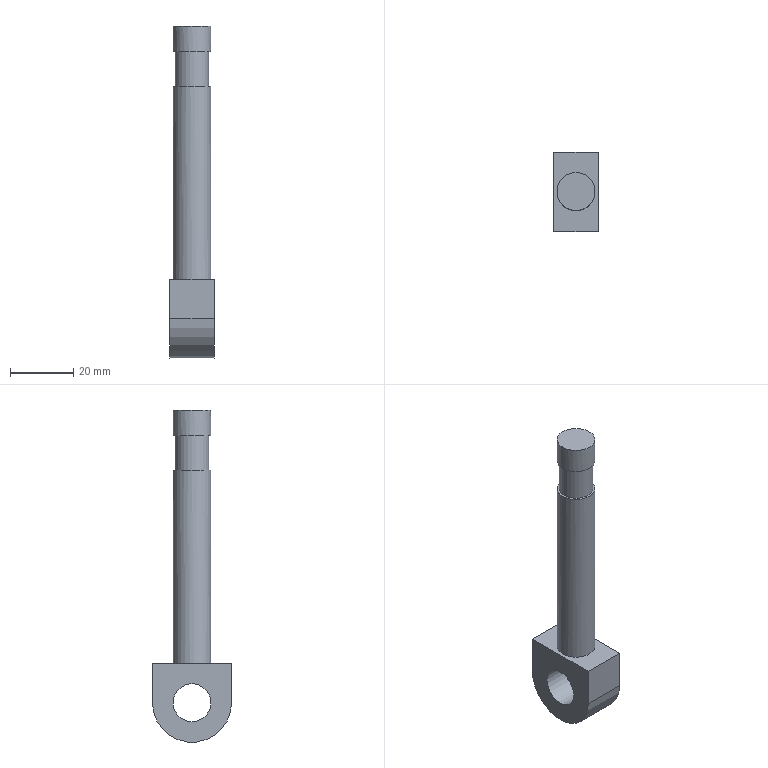Component | NX | HINGE_SCREW | 1 solid | 13 faces | box 14 x 25 x 105 mm | volume 15003 mm3 | plane 8 | cylinder 5 | commonest cylinder face diameters 12 x3 25 x1 10.579 x1
STEP:
#1=CARTESIAN_POINT('',(0.,0.,0.));
#2=DIRECTION('',(0.,0.,1.));
#3=DIRECTION('',(1.,0.,0.));
#4=AXIS2_PLACEMENT_3D('',#1,#2,#3);
#5=CARTESIAN_POINT('',(553.625,-108.409,-19.557));
#6=VERTEX_POINT('',#5);
#7=CARTESIAN_POINT('',(553.625,-108.409,-32.057));
#8=VERTEX_POINT('',#7);
#9=CARTESIAN_POINT('',(553.625,-108.409,-19.557));
#10=DIRECTION('',(0.,0.,-1.));
#11=VECTOR('',#10,1.);
#12=LINE('',#9,#11);
#13=CARTESIAN_POINT('',(567.625,-108.409,-19.557));
#14=DIRECTION('',(0.,1.,0.));
#15=DIRECTION('',(0.,0.,1.));
#16=AXIS2_PLACEMENT_3D('',#13,#14,#15);
#17=PLANE('',#16);
#18=CARTESIAN_POINT('',(0.,-14.));
#19=DIRECTION('',(-1.,0.));
#20=VECTOR('',#19,1.);
#21=LINE('',#18,#20);
#22=(GEOMETRIC_REPRESENTATION_CONTEXT(2)PARAMETRIC_REPRESENTATION_CONTEXT()REPRESENTATION_CONTEXT('',''));
#23=DEFINITIONAL_REPRESENTATION('',(#21),#22);
#24=PCURVE('',#17,#23);
#25=CARTESIAN_POINT('',(553.625,-95.909,-32.057));
#26=DIRECTION('',(1.,0.,0.));
#27=DIRECTION('',(0.,0.,-1.));
#28=AXIS2_PLACEMENT_3D('',#25,#26,#27);
#29=PLANE('',#28);
#30=CARTESIAN_POINT('',(-12.5,-12.5));
#31=DIRECTION('',(1.,0.));
#32=VECTOR('',#31,1.);
#33=LINE('',#30,#32);
#34=(GEOMETRIC_REPRESENTATION_CONTEXT(2)PARAMETRIC_REPRESENTATION_CONTEXT()REPRESENTATION_CONTEXT('',''));
#35=DEFINITIONAL_REPRESENTATION('',(#33),#34);
#36=PCURVE('',#29,#35);
#37=SURFACE_CURVE('',#12,(#24,#36),.PCURVE_S1.);
#38=EDGE_CURVE('',#6,#8,#37,.T.);
#39=ORIENTED_EDGE('',*,*,#38,.T.);
#40=CARTESIAN_POINT('',(567.625,-108.409,-32.057));
#41=VERTEX_POINT('',#40);
#42=CARTESIAN_POINT('',(567.625,-108.409,-32.057));
#43=DIRECTION('',(-1.,0.,0.));
#44=VECTOR('',#43,1.);
#45=LINE('',#42,#44);
#46=CARTESIAN_POINT('',(-12.5,0.));
#47=DIRECTION('',(0.,-1.));
#48=VECTOR('',#47,1.);
#49=LINE('',#46,#48);
#50=(GEOMETRIC_REPRESENTATION_CONTEXT(2)PARAMETRIC_REPRESENTATION_CONTEXT()REPRESENTATION_CONTEXT('',''));
#51=DEFINITIONAL_REPRESENTATION('',(#49),#50);
#52=PCURVE('',#17,#51);
#53=CARTESIAN_POINT('',(567.625,-95.909,-32.057));
#54=DIRECTION('',(-1.,0.,0.));
#55=DIRECTION('',(0.,0.,1.));
#56=AXIS2_PLACEMENT_3D('',#53,#54,#55);
#57=CYLINDRICAL_SURFACE('',#56,12.5);
#58=CARTESIAN_POINT('',(4.712,0.));
#59=DIRECTION('',(0.,1.));
#60=VECTOR('',#59,1.);
#61=LINE('',#58,#60);
#62=(GEOMETRIC_REPRESENTATION_CONTEXT(2)PARAMETRIC_REPRESENTATION_CONTEXT()REPRESENTATION_CONTEXT('',''));
#63=DEFINITIONAL_REPRESENTATION('',(#61),#62);
#64=PCURVE('',#57,#63);
#65=SURFACE_CURVE('',#45,(#52,#64),.PCURVE_S1.);
#66=EDGE_CURVE('',#41,#8,#65,.T.);
#67=ORIENTED_EDGE('',*,*,#66,.F.);
#68=CARTESIAN_POINT('',(567.625,-108.409,-19.557));
#69=VERTEX_POINT('',#68);
#70=CARTESIAN_POINT('',(567.625,-108.409,-19.557));
#71=DIRECTION('',(0.,0.,-1.));
#72=VECTOR('',#71,1.);
#73=LINE('',#70,#72);
#74=CARTESIAN_POINT('',(0.,0.));
#75=DIRECTION('',(-1.,0.));
#76=VECTOR('',#75,1.);
#77=LINE('',#74,#76);
#78=(GEOMETRIC_REPRESENTATION_CONTEXT(2)PARAMETRIC_REPRESENTATION_CONTEXT()REPRESENTATION_CONTEXT('',''));
#79=DEFINITIONAL_REPRESENTATION('',(#77),#78);
#80=PCURVE('',#17,#79);
#81=CARTESIAN_POINT('',(567.625,-95.909,-32.057));
#82=DIRECTION('',(1.,0.,0.));
#83=DIRECTION('',(0.,0.,-1.));
#84=AXIS2_PLACEMENT_3D('',#81,#82,#83);
#85=PLANE('',#84);
#86=CARTESIAN_POINT('',(-12.5,-12.5));
#87=DIRECTION('',(1.,0.));
#88=VECTOR('',#87,1.);
#89=LINE('',#86,#88);
#90=(GEOMETRIC_REPRESENTATION_CONTEXT(2)PARAMETRIC_REPRESENTATION_CONTEXT()REPRESENTATION_CONTEXT('',''));
#91=DEFINITIONAL_REPRESENTATION('',(#89),#90);
#92=PCURVE('',#85,#91);
#93=SURFACE_CURVE('',#73,(#80,#92),.PCURVE_S1.);
#94=EDGE_CURVE('',#69,#41,#93,.T.);
#95=ORIENTED_EDGE('',*,*,#94,.F.);
#96=CARTESIAN_POINT('',(567.625,-108.409,-19.557));
#97=DIRECTION('',(-1.,0.,0.));
#98=VECTOR('',#97,1.);
#99=LINE('',#96,#98);
#100=CARTESIAN_POINT('',(0.,0.));
#101=DIRECTION('',(0.,-1.));
#102=VECTOR('',#101,1.);
#103=LINE('',#100,#102);
#104=(GEOMETRIC_REPRESENTATION_CONTEXT(2)PARAMETRIC_REPRESENTATION_CONTEXT()REPRESENTATION_CONTEXT('',''));
#105=DEFINITIONAL_REPRESENTATION('',(#103),#104);
#106=PCURVE('',#17,#105);
#107=CARTESIAN_POINT('',(567.625,-83.409,-19.557));
#108=DIRECTION('',(0.,0.,-1.));
#109=DIRECTION('',(0.,1.,0.));
#110=AXIS2_PLACEMENT_3D('',#107,#108,#109);
#111=PLANE('',#110);
#112=CARTESIAN_POINT('',(-25.,0.));
#113=DIRECTION('',(0.,-1.));
#114=VECTOR('',#113,1.);
#115=LINE('',#112,#114);
#116=(GEOMETRIC_REPRESENTATION_CONTEXT(2)PARAMETRIC_REPRESENTATION_CONTEXT()REPRESENTATION_CONTEXT('',''));
#117=DEFINITIONAL_REPRESENTATION('',(#115),#116);
#118=PCURVE('',#111,#117);
#119=SURFACE_CURVE('',#99,(#106,#118),.PCURVE_S1.);
#120=EDGE_CURVE('',#69,#6,#119,.T.);
#121=ORIENTED_EDGE('',*,*,#120,.T.);
#122=EDGE_LOOP('',(#39,#67,#95,#121));
#123=FACE_BOUND('',#122,.T.);
#124=ADVANCED_FACE('',(#123),#17,.F.);
#125=CARTESIAN_POINT('',(553.625,-83.409,-32.057));
#126=VERTEX_POINT('',#125);
#127=CARTESIAN_POINT('',(553.625,-95.909,-32.057));
#128=DIRECTION('',(1.,0.,0.));
#129=DIRECTION('',(0.,1.,0.));
#130=AXIS2_PLACEMENT_3D('',#127,#128,#129);
#131=CIRCLE('',#130,12.5);
#132=CARTESIAN_POINT('',(7.854,14.));
#133=DIRECTION('',(-1.,0.));
#134=VECTOR('',#133,1.);
#135=LINE('',#132,#134);
#136=(GEOMETRIC_REPRESENTATION_CONTEXT(2)PARAMETRIC_REPRESENTATION_CONTEXT()REPRESENTATION_CONTEXT('',''));
#137=DEFINITIONAL_REPRESENTATION('',(#135),#136);
#138=PCURVE('',#57,#137);
#139=CARTESIAN_POINT('',(0.,0.));
#140=DIRECTION('',(0.,1.));
#141=AXIS2_PLACEMENT_2D('',#139,#140);
#142=CIRCLE('',#141,12.5);
#143=(GEOMETRIC_REPRESENTATION_CONTEXT(2)PARAMETRIC_REPRESENTATION_CONTEXT()REPRESENTATION_CONTEXT('',''));
#144=DEFINITIONAL_REPRESENTATION('',(#142),#143);
#145=PCURVE('',#29,#144);
#146=SURFACE_CURVE('',#131,(#138,#145),.PCURVE_S1.);
#147=EDGE_CURVE('',#8,#126,#146,.T.);
#148=ORIENTED_EDGE('',*,*,#147,.T.);
#149=CARTESIAN_POINT('',(567.625,-83.409,-32.057));
#150=VERTEX_POINT('',#149);
#151=CARTESIAN_POINT('',(567.625,-83.409,-32.057));
#152=DIRECTION('',(-1.,0.,0.));
#153=VECTOR('',#152,1.);
#154=LINE('',#151,#153);
#155=CARTESIAN_POINT('',(1.571,0.));
#156=DIRECTION('',(0.,1.));
#157=VECTOR('',#156,1.);
#158=LINE('',#155,#157);
#159=(GEOMETRIC_REPRESENTATION_CONTEXT(2)PARAMETRIC_REPRESENTATION_CONTEXT()REPRESENTATION_CONTEXT('',''));
#160=DEFINITIONAL_REPRESENTATION('',(#158),#159);
#161=PCURVE('',#57,#160);
#162=CARTESIAN_POINT('',(567.625,-83.409,-32.057));
#163=DIRECTION('',(0.,-1.,0.));
#164=DIRECTION('',(0.,0.,-1.));
#165=AXIS2_PLACEMENT_3D('',#162,#163,#164);
#166=PLANE('',#165);
#167=CARTESIAN_POINT('',(0.,0.));
#168=DIRECTION('',(0.,-1.));
#169=VECTOR('',#168,1.);
#170=LINE('',#167,#169);
#171=(GEOMETRIC_REPRESENTATION_CONTEXT(2)PARAMETRIC_REPRESENTATION_CONTEXT()REPRESENTATION_CONTEXT('',''));
#172=DEFINITIONAL_REPRESENTATION('',(#170),#171);
#173=PCURVE('',#166,#172);
#174=SURFACE_CURVE('',#154,(#161,#173),.PCURVE_S1.);
#175=EDGE_CURVE('',#150,#126,#174,.T.);
#176=ORIENTED_EDGE('',*,*,#175,.F.);
#177=CARTESIAN_POINT('',(567.625,-95.909,-32.057));
#178=DIRECTION('',(1.,0.,0.));
#179=DIRECTION('',(0.,1.,0.));
#180=AXIS2_PLACEMENT_3D('',#177,#178,#179);
#181=CIRCLE('',#180,12.5);
#182=CARTESIAN_POINT('',(7.854,0.));
#183=DIRECTION('',(-1.,0.));
#184=VECTOR('',#183,1.);
#185=LINE('',#182,#184);
#186=(GEOMETRIC_REPRESENTATION_CONTEXT(2)PARAMETRIC_REPRESENTATION_CONTEXT()REPRESENTATION_CONTEXT('',''));
#187=DEFINITIONAL_REPRESENTATION('',(#185),#186);
#188=PCURVE('',#57,#187);
#189=CARTESIAN_POINT('',(0.,0.));
#190=DIRECTION('',(0.,1.));
#191=AXIS2_PLACEMENT_2D('',#189,#190);
#192=CIRCLE('',#191,12.5);
#193=(GEOMETRIC_REPRESENTATION_CONTEXT(2)PARAMETRIC_REPRESENTATION_CONTEXT()REPRESENTATION_CONTEXT('',''));
#194=DEFINITIONAL_REPRESENTATION('',(#192),#193);
#195=PCURVE('',#85,#194);
#196=SURFACE_CURVE('',#181,(#188,#195),.PCURVE_S1.);
#197=EDGE_CURVE('',#41,#150,#196,.T.);
#198=ORIENTED_EDGE('',*,*,#197,.F.);
#199=ORIENTED_EDGE('',*,*,#66,.T.);
#200=EDGE_LOOP('',(#148,#176,#198,#199));
#201=FACE_BOUND('',#200,.T.);
#202=ADVANCED_FACE('',(#201),#57,.T.);
#203=CARTESIAN_POINT('',(553.625,-83.409,-19.557));
#204=VERTEX_POINT('',#203);
#205=CARTESIAN_POINT('',(553.625,-83.409,-32.057));
#206=DIRECTION('',(0.,0.,1.));
#207=VECTOR('',#206,1.);
#208=LINE('',#205,#207);
#209=CARTESIAN_POINT('',(0.,-14.));
#210=DIRECTION('',(-1.,0.));
#211=VECTOR('',#210,1.);
#212=LINE('',#209,#211);
#213=(GEOMETRIC_REPRESENTATION_CONTEXT(2)PARAMETRIC_REPRESENTATION_CONTEXT()REPRESENTATION_CONTEXT('',''));
#214=DEFINITIONAL_REPRESENTATION('',(#212),#213);
#215=PCURVE('',#166,#214);
#216=CARTESIAN_POINT('',(0.,12.5));
#217=DIRECTION('',(-1.,0.));
#218=VECTOR('',#217,1.);
#219=LINE('',#216,#218);
#220=(GEOMETRIC_REPRESENTATION_CONTEXT(2)PARAMETRIC_REPRESENTATION_CONTEXT()REPRESENTATION_CONTEXT('',''));
#221=DEFINITIONAL_REPRESENTATION('',(#219),#220);
#222=PCURVE('',#29,#221);
#223=SURFACE_CURVE('',#208,(#215,#222),.PCURVE_S1.);
#224=EDGE_CURVE('',#126,#204,#223,.T.);
#225=ORIENTED_EDGE('',*,*,#224,.T.);
#226=CARTESIAN_POINT('',(567.625,-83.409,-19.557));
#227=VERTEX_POINT('',#226);
#228=CARTESIAN_POINT('',(567.625,-83.409,-19.557));
#229=DIRECTION('',(-1.,0.,0.));
#230=VECTOR('',#229,1.);
#231=LINE('',#228,#230);
#232=CARTESIAN_POINT('',(-12.5,0.));
#233=DIRECTION('',(0.,-1.));
#234=VECTOR('',#233,1.);
#235=LINE('',#232,#234);
#236=(GEOMETRIC_REPRESENTATION_CONTEXT(2)PARAMETRIC_REPRESENTATION_CONTEXT()REPRESENTATION_CONTEXT('',''));
#237=DEFINITIONAL_REPRESENTATION('',(#235),#236);
#238=PCURVE('',#166,#237);
#239=CARTESIAN_POINT('',(0.,0.));
#240=DIRECTION('',(0.,-1.));
#241=VECTOR('',#240,1.);
#242=LINE('',#239,#241);
#243=(GEOMETRIC_REPRESENTATION_CONTEXT(2)PARAMETRIC_REPRESENTATION_CONTEXT()REPRESENTATION_CONTEXT('',''));
#244=DEFINITIONAL_REPRESENTATION('',(#242),#243);
#245=PCURVE('',#111,#244);
#246=SURFACE_CURVE('',#231,(#238,#245),.PCURVE_S1.);
#247=EDGE_CURVE('',#227,#204,#246,.T.);
#248=ORIENTED_EDGE('',*,*,#247,.F.);
#249=CARTESIAN_POINT('',(567.625,-83.409,-32.057));
#250=DIRECTION('',(0.,0.,1.));
#251=VECTOR('',#250,1.);
#252=LINE('',#249,#251);
#253=CARTESIAN_POINT('',(0.,0.));
#254=DIRECTION('',(-1.,0.));
#255=VECTOR('',#254,1.);
#256=LINE('',#253,#255);
#257=(GEOMETRIC_REPRESENTATION_CONTEXT(2)PARAMETRIC_REPRESENTATION_CONTEXT()REPRESENTATION_CONTEXT('',''));
#258=DEFINITIONAL_REPRESENTATION('',(#256),#257);
#259=PCURVE('',#166,#258);
#260=CARTESIAN_POINT('',(0.,12.5));
#261=DIRECTION('',(-1.,0.));
#262=VECTOR('',#261,1.);
#263=LINE('',#260,#262);
#264=(GEOMETRIC_REPRESENTATION_CONTEXT(2)PARAMETRIC_REPRESENTATION_CONTEXT()REPRESENTATION_CONTEXT('',''));
#265=DEFINITIONAL_REPRESENTATION('',(#263),#264);
#266=PCURVE('',#85,#265);
#267=SURFACE_CURVE('',#252,(#259,#266),.PCURVE_S1.);
#268=EDGE_CURVE('',#150,#227,#267,.T.);
#269=ORIENTED_EDGE('',*,*,#268,.F.);
#270=ORIENTED_EDGE('',*,*,#175,.T.);
#271=EDGE_LOOP('',(#225,#248,#269,#270));
#272=FACE_BOUND('',#271,.T.);
#273=ADVANCED_FACE('',(#272),#166,.F.);
#274=CARTESIAN_POINT('',(560.625,-89.909,-19.557));
#275=VERTEX_POINT('',#274);
#276=CARTESIAN_POINT('',(560.625,-95.909,-19.557));
#277=DIRECTION('',(0.,-0.,1.));
#278=DIRECTION('',(0.,1.,0.));
#279=AXIS2_PLACEMENT_3D('',#276,#277,#278);
#280=CIRCLE('',#279,6.);
#281=CARTESIAN_POINT('',(-6.5,-7.));
#282=CARTESIAN_POINT('',(-6.5,-17.392));
#283=CARTESIAN_POINT('',(-15.5,-12.196));
#284=CARTESIAN_POINT('',(-24.5,-7.));
#285=CARTESIAN_POINT('',(-15.5,-1.804));
#286=CARTESIAN_POINT('',(-6.5,3.392));
#287=CARTESIAN_POINT('',(-6.5,-7.));
#288=(BOUNDED_CURVE()B_SPLINE_CURVE(2,(#281,#282,#283,#284,#285,#286,#287),.UNSPECIFIED.,.T.,.F.)B_SPLINE_CURVE_WITH_KNOTS((1,2,2,2,2,1),(-2.094,0.,2.094,4.189,6.283,8.378),.UNSPECIFIED.)CURVE()GEOMETRIC_REPRESENTATION_ITEM()RATIONAL_B_SPLINE_CURVE((1.,0.5,1.,0.5,1.,0.5,1.))REPRESENTATION_ITEM(''));
#289=(GEOMETRIC_REPRESENTATION_CONTEXT(2)PARAMETRIC_REPRESENTATION_CONTEXT()REPRESENTATION_CONTEXT('',''));
#290=DEFINITIONAL_REPRESENTATION('',(#288),#289);
#291=PCURVE('',#111,#290);
#292=CARTESIAN_POINT('',(560.625,-95.909,60.443));
#293=DIRECTION('',(0.,0.,-1.));
#294=DIRECTION('',(0.,1.,0.));
#295=AXIS2_PLACEMENT_3D('',#292,#293,#294);
#296=CYLINDRICAL_SURFACE('',#295,6.);
#297=CARTESIAN_POINT('',(6.283,80.));
#298=DIRECTION('',(-1.,0.));
#299=VECTOR('',#298,1.);
#300=LINE('',#297,#299);
#301=(GEOMETRIC_REPRESENTATION_CONTEXT(2)PARAMETRIC_REPRESENTATION_CONTEXT()REPRESENTATION_CONTEXT('',''));
#302=DEFINITIONAL_REPRESENTATION('',(#300),#301);
#303=PCURVE('',#296,#302);
#304=SURFACE_CURVE('',#280,(#291,#303),.PCURVE_S1.);
#305=EDGE_CURVE('',#275,#275,#304,.T.);
#306=ORIENTED_EDGE('',*,*,#305,.F.);
#307=EDGE_LOOP('',(#306));
#308=FACE_BOUND('',#307,.T.);
#309=CARTESIAN_POINT('',(553.625,-83.409,-19.557));
#310=DIRECTION('',(0.,-1.,-0.));
#311=VECTOR('',#310,1.);
#312=LINE('',#309,#311);
#313=CARTESIAN_POINT('',(0.,-14.));
#314=DIRECTION('',(-1.,0.));
#315=VECTOR('',#314,1.);
#316=LINE('',#313,#315);
#317=(GEOMETRIC_REPRESENTATION_CONTEXT(2)PARAMETRIC_REPRESENTATION_CONTEXT()REPRESENTATION_CONTEXT('',''));
#318=DEFINITIONAL_REPRESENTATION('',(#316),#317);
#319=PCURVE('',#111,#318);
#320=CARTESIAN_POINT('',(-12.5,12.5));
#321=DIRECTION('',(0.,-1.));
#322=VECTOR('',#321,1.);
#323=LINE('',#320,#322);
#324=(GEOMETRIC_REPRESENTATION_CONTEXT(2)PARAMETRIC_REPRESENTATION_CONTEXT()REPRESENTATION_CONTEXT('',''));
#325=DEFINITIONAL_REPRESENTATION('',(#323),#324);
#326=PCURVE('',#29,#325);
#327=SURFACE_CURVE('',#312,(#319,#326),.PCURVE_S1.);
#328=EDGE_CURVE('',#204,#6,#327,.T.);
#329=ORIENTED_EDGE('',*,*,#328,.T.);
#330=ORIENTED_EDGE('',*,*,#120,.F.);
#331=CARTESIAN_POINT('',(567.625,-83.409,-19.557));
#332=DIRECTION('',(0.,-1.,-0.));
#333=VECTOR('',#332,1.);
#334=LINE('',#331,#333);
#335=CARTESIAN_POINT('',(0.,0.));
#336=DIRECTION('',(-1.,0.));
#337=VECTOR('',#336,1.);
#338=LINE('',#335,#337);
#339=(GEOMETRIC_REPRESENTATION_CONTEXT(2)PARAMETRIC_REPRESENTATION_CONTEXT()REPRESENTATION_CONTEXT('',''));
#340=DEFINITIONAL_REPRESENTATION('',(#338),#339);
#341=PCURVE('',#111,#340);
#342=CARTESIAN_POINT('',(-12.5,12.5));
#343=DIRECTION('',(0.,-1.));
#344=VECTOR('',#343,1.);
#345=LINE('',#342,#344);
#346=(GEOMETRIC_REPRESENTATION_CONTEXT(2)PARAMETRIC_REPRESENTATION_CONTEXT()REPRESENTATION_CONTEXT('',''));
#347=DEFINITIONAL_REPRESENTATION('',(#345),#346);
#348=PCURVE('',#85,#347);
#349=SURFACE_CURVE('',#334,(#341,#348),.PCURVE_S1.);
#350=EDGE_CURVE('',#227,#69,#349,.T.);
#351=ORIENTED_EDGE('',*,*,#350,.F.);
#352=ORIENTED_EDGE('',*,*,#247,.T.);
#353=EDGE_LOOP('',(#329,#330,#351,#352));
#354=FACE_BOUND('',#353,.T.);
#355=ADVANCED_FACE('',(#308,#354),#111,.F.);
#356=CARTESIAN_POINT('',(567.625,-89.909,-32.057));
#357=VERTEX_POINT('',#356);
#358=CARTESIAN_POINT('',(567.625,-95.909,-32.057));
#359=DIRECTION('',(1.,0.,0.));
#360=DIRECTION('',(0.,1.,0.));
#361=AXIS2_PLACEMENT_3D('',#358,#359,#360);
#362=CIRCLE('',#361,6.);
#363=CARTESIAN_POINT('',(567.625,-95.909,-32.057));
#364=DIRECTION('',(-1.,0.,0.));
#365=DIRECTION('',(0.,0.,1.));
#366=AXIS2_PLACEMENT_3D('',#363,#364,#365);
#367=CYLINDRICAL_SURFACE('',#366,6.);
#368=CARTESIAN_POINT('',(7.854,0.));
#369=DIRECTION('',(-1.,0.));
#370=VECTOR('',#369,1.);
#371=LINE('',#368,#370);
#372=(GEOMETRIC_REPRESENTATION_CONTEXT(2)PARAMETRIC_REPRESENTATION_CONTEXT()REPRESENTATION_CONTEXT('',''));
#373=DEFINITIONAL_REPRESENTATION('',(#371),#372);
#374=PCURVE('',#367,#373);
#375=CARTESIAN_POINT('',(0.,0.));
#376=DIRECTION('',(0.,1.));
#377=AXIS2_PLACEMENT_2D('',#375,#376);
#378=CIRCLE('',#377,6.);
#379=(GEOMETRIC_REPRESENTATION_CONTEXT(2)PARAMETRIC_REPRESENTATION_CONTEXT()REPRESENTATION_CONTEXT('',''));
#380=DEFINITIONAL_REPRESENTATION('',(#378),#379);
#381=PCURVE('',#85,#380);
#382=SURFACE_CURVE('',#362,(#374,#381),.PCURVE_S1.);
#383=EDGE_CURVE('',#357,#357,#382,.T.);
#384=ORIENTED_EDGE('',*,*,#383,.F.);
#385=CARTESIAN_POINT('',(553.625,-89.909,-32.057));
#386=VERTEX_POINT('',#385);
#387=CARTESIAN_POINT('',(567.625,-89.909,-32.057));
#388=CARTESIAN_POINT('',(553.625,-89.909,-32.057));
#389=B_SPLINE_CURVE_WITH_KNOTS('',1,(#387,#388),.UNSPECIFIED.,.F.,.F.,(2,2),(0.,14.),.PIECEWISE_BEZIER_KNOTS.);
#390=CARTESIAN_POINT('',(7.854,0.));
#391=DIRECTION('',(0.,1.));
#392=VECTOR('',#391,1.);
#393=LINE('',#390,#392);
#394=(GEOMETRIC_REPRESENTATION_CONTEXT(2)PARAMETRIC_REPRESENTATION_CONTEXT()REPRESENTATION_CONTEXT('',''));
#395=DEFINITIONAL_REPRESENTATION('',(#393),#394);
#396=PCURVE('',#367,#395);
#397=CARTESIAN_POINT('',(1.571,0.));
#398=DIRECTION('',(0.,1.));
#399=VECTOR('',#398,1.);
#400=LINE('',#397,#399);
#401=(GEOMETRIC_REPRESENTATION_CONTEXT(2)PARAMETRIC_REPRESENTATION_CONTEXT()REPRESENTATION_CONTEXT('',''));
#402=DEFINITIONAL_REPRESENTATION('',(#400),#401);
#403=PCURVE('',#367,#402);
#404=SEAM_CURVE('',#389,(#396,#403),.PCURVE_S1.);
#405=EDGE_CURVE('',#357,#386,#404,.T.);
#406=ORIENTED_EDGE('',*,*,#405,.T.);
#407=CARTESIAN_POINT('',(553.625,-95.909,-32.057));
#408=DIRECTION('',(1.,0.,0.));
#409=DIRECTION('',(0.,1.,0.));
#410=AXIS2_PLACEMENT_3D('',#407,#408,#409);
#411=CIRCLE('',#410,6.);
#412=CARTESIAN_POINT('',(7.854,14.));
#413=DIRECTION('',(-1.,0.));
#414=VECTOR('',#413,1.);
#415=LINE('',#412,#414);
#416=(GEOMETRIC_REPRESENTATION_CONTEXT(2)PARAMETRIC_REPRESENTATION_CONTEXT()REPRESENTATION_CONTEXT('',''));
#417=DEFINITIONAL_REPRESENTATION('',(#415),#416);
#418=PCURVE('',#367,#417);
#419=CARTESIAN_POINT('',(0.,0.));
#420=DIRECTION('',(0.,1.));
#421=AXIS2_PLACEMENT_2D('',#419,#420);
#422=CIRCLE('',#421,6.);
#423=(GEOMETRIC_REPRESENTATION_CONTEXT(2)PARAMETRIC_REPRESENTATION_CONTEXT()REPRESENTATION_CONTEXT('',''));
#424=DEFINITIONAL_REPRESENTATION('',(#422),#423);
#425=PCURVE('',#29,#424);
#426=SURFACE_CURVE('',#411,(#418,#425),.PCURVE_S1.);
#427=EDGE_CURVE('',#386,#386,#426,.T.);
#428=ORIENTED_EDGE('',*,*,#427,.T.);
#429=ORIENTED_EDGE('',*,*,#405,.F.);
#430=EDGE_LOOP('',(#384,#406,#428,#429));
#431=FACE_BOUND('',#430,.F.);
#432=ADVANCED_FACE('',(#431),#367,.F.);
#433=ORIENTED_EDGE('',*,*,#94,.T.);
#434=ORIENTED_EDGE('',*,*,#197,.T.);
#435=ORIENTED_EDGE('',*,*,#268,.T.);
#436=ORIENTED_EDGE('',*,*,#350,.T.);
#437=EDGE_LOOP('',(#433,#434,#435,#436));
#438=FACE_BOUND('',#437,.T.);
#439=ORIENTED_EDGE('',*,*,#383,.F.);
#440=EDGE_LOOP('',(#439));
#441=FACE_BOUND('',#440,.T.);
#442=ADVANCED_FACE('',(#438,#441),#85,.T.);
#443=ORIENTED_EDGE('',*,*,#38,.F.);
#444=ORIENTED_EDGE('',*,*,#328,.F.);
#445=ORIENTED_EDGE('',*,*,#224,.F.);
#446=ORIENTED_EDGE('',*,*,#147,.F.);
#447=EDGE_LOOP('',(#443,#444,#445,#446));
#448=FACE_BOUND('',#447,.T.);
#449=ORIENTED_EDGE('',*,*,#427,.T.);
#450=EDGE_LOOP('',(#449));
#451=FACE_BOUND('',#450,.T.);
#452=ADVANCED_FACE('',(#448,#451),#29,.F.);
#453=CARTESIAN_POINT('',(554.625,-95.909,41.443));
#454=VERTEX_POINT('',#453);
#455=CARTESIAN_POINT('',(560.625,-89.909,41.443));
#456=VERTEX_POINT('',#455);
#457=CARTESIAN_POINT('',(560.625,-95.909,41.443));
#458=DIRECTION('',(0.,0.,-1.));
#459=DIRECTION('',(-1.,0.,0.));
#460=AXIS2_PLACEMENT_3D('',#457,#458,#459);
#461=CIRCLE('',#460,6.);
#462=CARTESIAN_POINT('',(4.712,19.));
#463=DIRECTION('',(1.,0.));
#464=VECTOR('',#463,1.);
#465=LINE('',#462,#464);
#466=(GEOMETRIC_REPRESENTATION_CONTEXT(2)PARAMETRIC_REPRESENTATION_CONTEXT()REPRESENTATION_CONTEXT('',''));
#467=DEFINITIONAL_REPRESENTATION('',(#465),#466);
#468=PCURVE('',#296,#467);
#469=CARTESIAN_POINT('',(560.625,-95.909,41.443));
#470=DIRECTION('',(0.,0.,-1.));
#471=DIRECTION('',(-1.,0.,0.));
#472=AXIS2_PLACEMENT_3D('',#469,#470,#471);
#473=PLANE('',#472);
#474=CARTESIAN_POINT('',(0.,0.));
#475=DIRECTION('',(1.,0.));
#476=AXIS2_PLACEMENT_2D('',#474,#475);
#477=CIRCLE('',#476,6.);
#478=(GEOMETRIC_REPRESENTATION_CONTEXT(2)PARAMETRIC_REPRESENTATION_CONTEXT()REPRESENTATION_CONTEXT('',''));
#479=DEFINITIONAL_REPRESENTATION('',(#477),#478);
#480=PCURVE('',#473,#479);
#481=SURFACE_CURVE('',#461,(#468,#480),.PCURVE_S1.);
#482=EDGE_CURVE('',#454,#456,#481,.T.);
#483=ORIENTED_EDGE('',*,*,#482,.T.);
#484=CARTESIAN_POINT('',(560.625,-89.909,41.443));
#485=CARTESIAN_POINT('',(560.625,-89.909,-19.557));
#486=B_SPLINE_CURVE_WITH_KNOTS('',1,(#484,#485),.UNSPECIFIED.,.F.,.F.,(2,2),(19.,80.),.PIECEWISE_BEZIER_KNOTS.);
#487=CARTESIAN_POINT('',(6.283,0.));
#488=DIRECTION('',(0.,1.));
#489=VECTOR('',#488,1.);
#490=LINE('',#487,#489);
#491=(GEOMETRIC_REPRESENTATION_CONTEXT(2)PARAMETRIC_REPRESENTATION_CONTEXT()REPRESENTATION_CONTEXT('',''));
#492=DEFINITIONAL_REPRESENTATION('',(#490),#491);
#493=PCURVE('',#296,#492);
#494=CARTESIAN_POINT('',(0.,0.));
#495=DIRECTION('',(0.,1.));
#496=VECTOR('',#495,1.);
#497=LINE('',#494,#496);
#498=(GEOMETRIC_REPRESENTATION_CONTEXT(2)PARAMETRIC_REPRESENTATION_CONTEXT()REPRESENTATION_CONTEXT('',''));
#499=DEFINITIONAL_REPRESENTATION('',(#497),#498);
#500=PCURVE('',#296,#499);
#501=SEAM_CURVE('',#486,(#493,#500),.PCURVE_S1.);
#502=EDGE_CURVE('',#456,#275,#501,.T.);
#503=ORIENTED_EDGE('',*,*,#502,.T.);
#504=ORIENTED_EDGE('',*,*,#305,.T.);
#505=ORIENTED_EDGE('',*,*,#502,.F.);
#506=CARTESIAN_POINT('',(560.625,-95.909,41.443));
#507=DIRECTION('',(0.,0.,-1.));
#508=DIRECTION('',(-1.,0.,0.));
#509=AXIS2_PLACEMENT_3D('',#506,#507,#508);
#510=CIRCLE('',#509,6.);
#511=CARTESIAN_POINT('',(-1.571,19.));
#512=DIRECTION('',(1.,0.));
#513=VECTOR('',#512,1.);
#514=LINE('',#511,#513);
#515=(GEOMETRIC_REPRESENTATION_CONTEXT(2)PARAMETRIC_REPRESENTATION_CONTEXT()REPRESENTATION_CONTEXT('',''));
#516=DEFINITIONAL_REPRESENTATION('',(#514),#515);
#517=PCURVE('',#296,#516);
#518=CARTESIAN_POINT('',(0.,0.));
#519=DIRECTION('',(1.,0.));
#520=AXIS2_PLACEMENT_2D('',#518,#519);
#521=CIRCLE('',#520,6.);
#522=(GEOMETRIC_REPRESENTATION_CONTEXT(2)PARAMETRIC_REPRESENTATION_CONTEXT()REPRESENTATION_CONTEXT('',''));
#523=DEFINITIONAL_REPRESENTATION('',(#521),#522);
#524=PCURVE('',#473,#523);
#525=SURFACE_CURVE('',#510,(#517,#524),.PCURVE_S1.);
#526=EDGE_CURVE('',#456,#454,#525,.T.);
#527=ORIENTED_EDGE('',*,*,#526,.T.);
#528=EDGE_LOOP('',(#483,#503,#504,#505,#527));
#529=FACE_BOUND('',#528,.T.);
#530=ADVANCED_FACE('',(#529),#296,.T.);
#531=CARTESIAN_POINT('',(565.914,-95.909,52.243));
#532=VERTEX_POINT('',#531);
#533=CARTESIAN_POINT('',(560.625,-95.909,52.243));
#534=DIRECTION('',(0.,0.,1.));
#535=DIRECTION('',(1.,0.,0.));
#536=AXIS2_PLACEMENT_3D('',#533,#534,#535);
#537=CIRCLE('',#536,5.29);
#538=CARTESIAN_POINT('',(560.625,-95.909,52.243));
#539=DIRECTION('',(0.,0.,1.));
#540=DIRECTION('',(1.,0.,0.));
#541=AXIS2_PLACEMENT_3D('',#538,#539,#540);
#542=PLANE('',#541);
#543=CARTESIAN_POINT('',(0.,0.));
#544=DIRECTION('',(1.,0.));
#545=AXIS2_PLACEMENT_2D('',#543,#544);
#546=CIRCLE('',#545,5.29);
#547=(GEOMETRIC_REPRESENTATION_CONTEXT(2)PARAMETRIC_REPRESENTATION_CONTEXT()REPRESENTATION_CONTEXT('',''));
#548=DEFINITIONAL_REPRESENTATION('',(#546),#547);
#549=PCURVE('',#542,#548);
#550=CARTESIAN_POINT('',(560.625,-95.909,41.443));
#551=DIRECTION('',(0.,0.,1.));
#552=DIRECTION('',(1.,0.,0.));
#553=AXIS2_PLACEMENT_3D('',#550,#551,#552);
#554=CYLINDRICAL_SURFACE('',#553,5.29);
#555=CARTESIAN_POINT('',(0.,10.8));
#556=DIRECTION('',(1.,0.));
#557=VECTOR('',#556,1.);
#558=LINE('',#555,#557);
#559=(GEOMETRIC_REPRESENTATION_CONTEXT(2)PARAMETRIC_REPRESENTATION_CONTEXT()REPRESENTATION_CONTEXT('',''));
#560=DEFINITIONAL_REPRESENTATION('',(#558),#559);
#561=PCURVE('',#554,#560);
#562=SURFACE_CURVE('',#537,(#549,#561),.PCURVE_S1.);
#563=EDGE_CURVE('',#532,#532,#562,.T.);
#564=ORIENTED_EDGE('',*,*,#563,.T.);
#565=EDGE_LOOP('',(#564));
#566=FACE_BOUND('',#565,.T.);
#567=CARTESIAN_POINT('',(566.625,-95.909,52.243));
#568=VERTEX_POINT('',#567);
#569=CARTESIAN_POINT('',(560.625,-89.909,52.243));
#570=VERTEX_POINT('',#569);
#571=CARTESIAN_POINT('',(560.625,-95.909,52.243));
#572=DIRECTION('',(0.,0.,1.));
#573=DIRECTION('',(1.,0.,0.));
#574=AXIS2_PLACEMENT_3D('',#571,#572,#573);
#575=CIRCLE('',#574,6.);
#576=CARTESIAN_POINT('',(0.,0.));
#577=DIRECTION('',(1.,0.));
#578=AXIS2_PLACEMENT_2D('',#576,#577);
#579=CIRCLE('',#578,6.);
#580=(GEOMETRIC_REPRESENTATION_CONTEXT(2)PARAMETRIC_REPRESENTATION_CONTEXT()REPRESENTATION_CONTEXT('',''));
#581=DEFINITIONAL_REPRESENTATION('',(#579),#580);
#582=PCURVE('',#542,#581);
#583=CARTESIAN_POINT('',(560.625,-95.909,60.443));
#584=DIRECTION('',(0.,0.,-1.));
#585=DIRECTION('',(0.,1.,0.));
#586=AXIS2_PLACEMENT_3D('',#583,#584,#585);
#587=CYLINDRICAL_SURFACE('',#586,6.);
#588=CARTESIAN_POINT('',(1.571,8.2));
#589=DIRECTION('',(-1.,0.));
#590=VECTOR('',#589,1.);
#591=LINE('',#588,#590);
#592=(GEOMETRIC_REPRESENTATION_CONTEXT(2)PARAMETRIC_REPRESENTATION_CONTEXT()REPRESENTATION_CONTEXT('',''));
#593=DEFINITIONAL_REPRESENTATION('',(#591),#592);
#594=PCURVE('',#587,#593);
#595=SURFACE_CURVE('',#575,(#582,#594),.PCURVE_S1.);
#596=EDGE_CURVE('',#568,#570,#595,.T.);
#597=ORIENTED_EDGE('',*,*,#596,.F.);
#598=CARTESIAN_POINT('',(560.625,-95.909,52.243));
#599=DIRECTION('',(0.,0.,1.));
#600=DIRECTION('',(1.,0.,0.));
#601=AXIS2_PLACEMENT_3D('',#598,#599,#600);
#602=CIRCLE('',#601,6.);
#603=CARTESIAN_POINT('',(0.,0.));
#604=DIRECTION('',(1.,0.));
#605=AXIS2_PLACEMENT_2D('',#603,#604);
#606=CIRCLE('',#605,6.);
#607=(GEOMETRIC_REPRESENTATION_CONTEXT(2)PARAMETRIC_REPRESENTATION_CONTEXT()REPRESENTATION_CONTEXT('',''));
#608=DEFINITIONAL_REPRESENTATION('',(#606),#607);
#609=PCURVE('',#542,#608);
#610=CARTESIAN_POINT('',(7.854,8.2));
#611=DIRECTION('',(-1.,0.));
#612=VECTOR('',#611,1.);
#613=LINE('',#610,#612);
#614=(GEOMETRIC_REPRESENTATION_CONTEXT(2)PARAMETRIC_REPRESENTATION_CONTEXT()REPRESENTATION_CONTEXT('',''));
#615=DEFINITIONAL_REPRESENTATION('',(#613),#614);
#616=PCURVE('',#587,#615);
#617=SURFACE_CURVE('',#602,(#609,#616),.PCURVE_S1.);
#618=EDGE_CURVE('',#570,#568,#617,.T.);
#619=ORIENTED_EDGE('',*,*,#618,.F.);
#620=EDGE_LOOP('',(#597,#619));
#621=FACE_BOUND('',#620,.T.);
#622=ADVANCED_FACE('',(#566,#621),#542,.F.);
#623=CARTESIAN_POINT('',(565.914,-95.909,41.443));
#624=VERTEX_POINT('',#623);
#625=CARTESIAN_POINT('',(560.625,-95.909,41.443));
#626=DIRECTION('',(0.,0.,-1.));
#627=DIRECTION('',(1.,0.,0.));
#628=AXIS2_PLACEMENT_3D('',#625,#626,#627);
#629=CIRCLE('',#628,5.29);
#630=CARTESIAN_POINT('',(0.,0.));
#631=DIRECTION('',(-1.,0.));
#632=AXIS2_PLACEMENT_2D('',#630,#631);
#633=CIRCLE('',#632,5.29);
#634=(GEOMETRIC_REPRESENTATION_CONTEXT(2)PARAMETRIC_REPRESENTATION_CONTEXT()REPRESENTATION_CONTEXT('',''));
#635=DEFINITIONAL_REPRESENTATION('',(#633),#634);
#636=PCURVE('',#473,#635);
#637=CARTESIAN_POINT('',(6.283,0.));
#638=DIRECTION('',(-1.,0.));
#639=VECTOR('',#638,1.);
#640=LINE('',#637,#639);
#641=(GEOMETRIC_REPRESENTATION_CONTEXT(2)PARAMETRIC_REPRESENTATION_CONTEXT()REPRESENTATION_CONTEXT('',''));
#642=DEFINITIONAL_REPRESENTATION('',(#640),#641);
#643=PCURVE('',#554,#642);
#644=SURFACE_CURVE('',#629,(#636,#643),.PCURVE_S1.);
#645=EDGE_CURVE('',#624,#624,#644,.T.);
#646=ORIENTED_EDGE('',*,*,#645,.T.);
#647=EDGE_LOOP('',(#646));
#648=FACE_BOUND('',#647,.T.);
#649=ORIENTED_EDGE('',*,*,#482,.F.);
#650=ORIENTED_EDGE('',*,*,#526,.F.);
#651=EDGE_LOOP('',(#649,#650));
#652=FACE_BOUND('',#651,.T.);
#653=ADVANCED_FACE('',(#648,#652),#473,.F.);
#654=ORIENTED_EDGE('',*,*,#563,.F.);
#655=CARTESIAN_POINT('',(565.914,-95.909,41.443));
#656=CARTESIAN_POINT('',(565.914,-95.909,52.243));
#657=B_SPLINE_CURVE_WITH_KNOTS('',1,(#655,#656),.UNSPECIFIED.,.F.,.F.,(2,2),(0.,10.8),.PIECEWISE_BEZIER_KNOTS.);
#658=CARTESIAN_POINT('',(0.,0.));
#659=DIRECTION('',(0.,1.));
#660=VECTOR('',#659,1.);
#661=LINE('',#658,#660);
#662=(GEOMETRIC_REPRESENTATION_CONTEXT(2)PARAMETRIC_REPRESENTATION_CONTEXT()REPRESENTATION_CONTEXT('',''));
#663=DEFINITIONAL_REPRESENTATION('',(#661),#662);
#664=PCURVE('',#554,#663);
#665=CARTESIAN_POINT('',(6.283,0.));
#666=DIRECTION('',(0.,1.));
#667=VECTOR('',#666,1.);
#668=LINE('',#665,#667);
#669=(GEOMETRIC_REPRESENTATION_CONTEXT(2)PARAMETRIC_REPRESENTATION_CONTEXT()REPRESENTATION_CONTEXT('',''));
#670=DEFINITIONAL_REPRESENTATION('',(#668),#669);
#671=PCURVE('',#554,#670);
#672=SEAM_CURVE('',#657,(#664,#671),.PCURVE_S1.);
#673=EDGE_CURVE('',#624,#532,#672,.T.);
#674=ORIENTED_EDGE('',*,*,#673,.F.);
#675=ORIENTED_EDGE('',*,*,#645,.F.);
#676=ORIENTED_EDGE('',*,*,#673,.T.);
#677=EDGE_LOOP('',(#654,#674,#675,#676));
#678=FACE_BOUND('',#677,.T.);
#679=ADVANCED_FACE('',(#678),#554,.T.);
#680=CARTESIAN_POINT('',(560.625,-89.909,60.443));
#681=VERTEX_POINT('',#680);
#682=CARTESIAN_POINT('',(560.625,-95.909,60.443));
#683=DIRECTION('',(0.,-0.,1.));
#684=DIRECTION('',(0.,1.,0.));
#685=AXIS2_PLACEMENT_3D('',#682,#683,#684);
#686=CIRCLE('',#685,6.);
#687=CARTESIAN_POINT('',(560.625,-95.909,60.443));
#688=DIRECTION('',(0.,-0.,1.));
#689=DIRECTION('',(0.,-1.,-0.));
#690=AXIS2_PLACEMENT_3D('',#687,#688,#689);
#691=PLANE('',#690);
#692=CARTESIAN_POINT('',(0.,0.));
#693=DIRECTION('',(-1.,0.));
#694=AXIS2_PLACEMENT_2D('',#692,#693);
#695=CIRCLE('',#694,6.);
#696=(GEOMETRIC_REPRESENTATION_CONTEXT(2)PARAMETRIC_REPRESENTATION_CONTEXT()REPRESENTATION_CONTEXT('',''));
#697=DEFINITIONAL_REPRESENTATION('',(#695),#696);
#698=PCURVE('',#691,#697);
#699=CARTESIAN_POINT('',(6.283,0.));
#700=DIRECTION('',(-1.,0.));
#701=VECTOR('',#700,1.);
#702=LINE('',#699,#701);
#703=(GEOMETRIC_REPRESENTATION_CONTEXT(2)PARAMETRIC_REPRESENTATION_CONTEXT()REPRESENTATION_CONTEXT('',''));
#704=DEFINITIONAL_REPRESENTATION('',(#702),#703);
#705=PCURVE('',#587,#704);
#706=SURFACE_CURVE('',#686,(#698,#705),.PCURVE_S1.);
#707=EDGE_CURVE('',#681,#681,#706,.T.);
#708=ORIENTED_EDGE('',*,*,#707,.T.);
#709=EDGE_LOOP('',(#708));
#710=FACE_BOUND('',#709,.T.);
#711=ADVANCED_FACE('',(#710),#691,.T.);
#712=ORIENTED_EDGE('',*,*,#596,.T.);
#713=CARTESIAN_POINT('',(560.625,-89.909,60.443));
#714=CARTESIAN_POINT('',(560.625,-89.909,52.243));
#715=B_SPLINE_CURVE_WITH_KNOTS('',1,(#713,#714),.UNSPECIFIED.,.F.,.F.,(2,2),(0.,8.2),.PIECEWISE_BEZIER_KNOTS.);
#716=CARTESIAN_POINT('',(0.,0.));
#717=DIRECTION('',(0.,1.));
#718=VECTOR('',#717,1.);
#719=LINE('',#716,#718);
#720=(GEOMETRIC_REPRESENTATION_CONTEXT(2)PARAMETRIC_REPRESENTATION_CONTEXT()REPRESENTATION_CONTEXT('',''));
#721=DEFINITIONAL_REPRESENTATION('',(#719),#720);
#722=PCURVE('',#587,#721);
#723=CARTESIAN_POINT('',(6.283,0.));
#724=DIRECTION('',(0.,1.));
#725=VECTOR('',#724,1.);
#726=LINE('',#723,#725);
#727=(GEOMETRIC_REPRESENTATION_CONTEXT(2)PARAMETRIC_REPRESENTATION_CONTEXT()REPRESENTATION_CONTEXT('',''));
#728=DEFINITIONAL_REPRESENTATION('',(#726),#727);
#729=PCURVE('',#587,#728);
#730=SEAM_CURVE('',#715,(#722,#729),.PCURVE_S1.);
#731=EDGE_CURVE('',#681,#570,#730,.T.);
#732=ORIENTED_EDGE('',*,*,#731,.F.);
#733=ORIENTED_EDGE('',*,*,#707,.F.);
#734=ORIENTED_EDGE('',*,*,#731,.T.);
#735=ORIENTED_EDGE('',*,*,#618,.T.);
#736=EDGE_LOOP('',(#712,#732,#733,#734,#735));
#737=FACE_BOUND('',#736,.T.);
#738=ADVANCED_FACE('',(#737),#587,.T.);
#739=CLOSED_SHELL('',(#124,#202,#273,#355,#432,#442,#452,#530,#622,#653,#679,#711,#738));
#740=MANIFOLD_SOLID_BREP('',#739);
#741=(LENGTH_UNIT()NAMED_UNIT(*)SI_UNIT(.MILLI.,.METRE.));
#742=UNCERTAINTY_MEASURE_WITH_UNIT(LENGTH_MEASURE(0.000005),#741,'','');
#743=(NAMED_UNIT(*)PLANE_ANGLE_UNIT()SI_UNIT($,.RADIAN.));
#744=(NAMED_UNIT(*)SI_UNIT($,.STERADIAN.)SOLID_ANGLE_UNIT());
#745=(GEOMETRIC_REPRESENTATION_CONTEXT(3)GLOBAL_UNCERTAINTY_ASSIGNED_CONTEXT((#742))GLOBAL_UNIT_ASSIGNED_CONTEXT((#741,#743,#744))REPRESENTATION_CONTEXT('',''));
#746=ADVANCED_BREP_SHAPE_REPRESENTATION('',(#4,#740),#745);